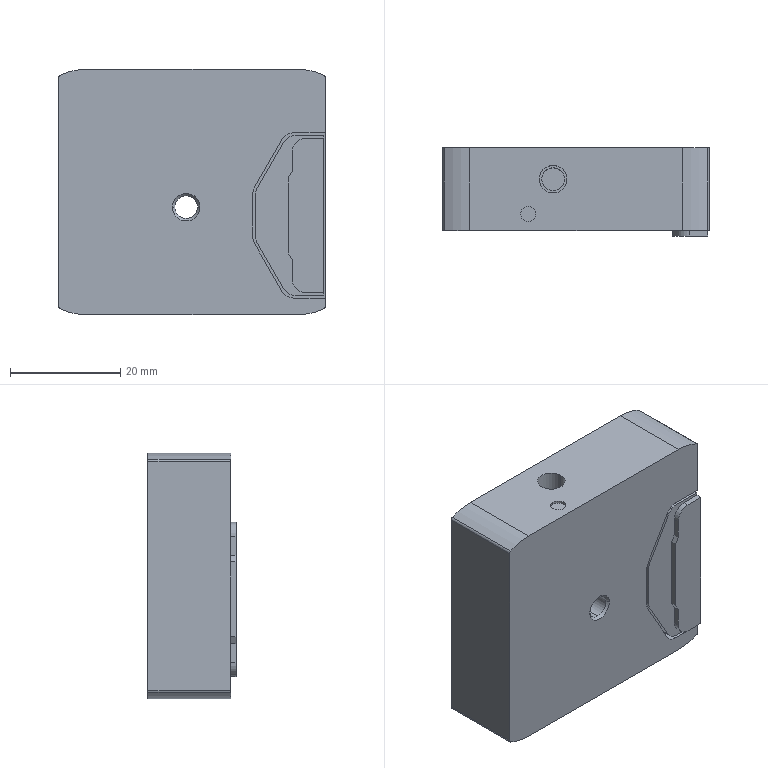Component | SolidWorks | DGC-18-280-G-PPV-A-1_HI_532446 DGC-18-G---(0DL)_1-1 | 1 solid | 104 faces | volume 31056 mm3 | cylinder 46 | plane 44 | cone 14 | commonest cylinder face diameters 5 x14 2 x10 3.242 x6 4.134 x4 21.6 x4 1 x4 2.8 x2 4.2 x2